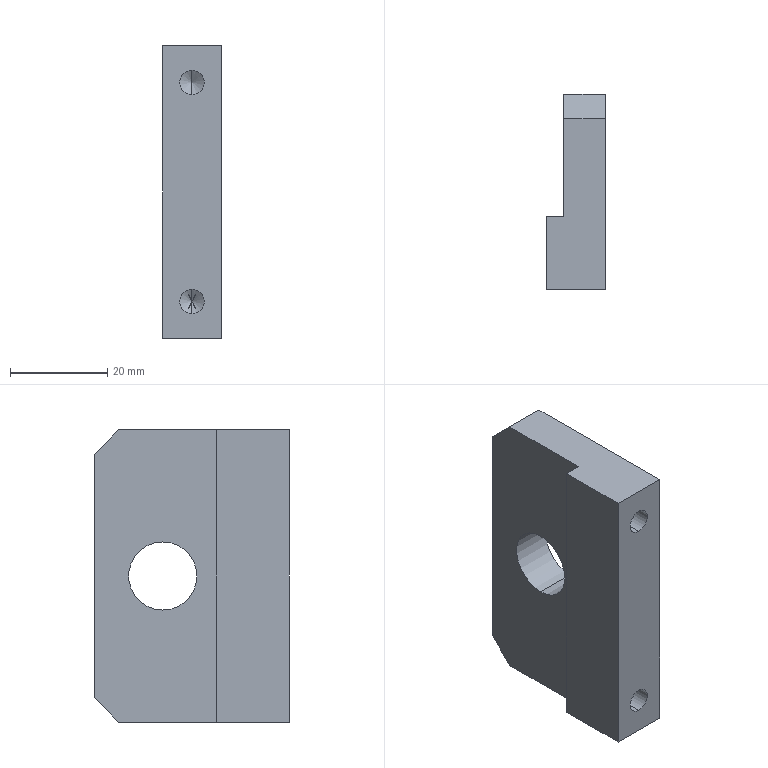Component | SolidWorks | OT-0100-009(TrunnionSeat)-1 | 1 solid | 20 faces | box 12 x 40 x 60 mm | volume 21499 mm3 | plane 10 | cylinder 6 | cone 4 | commonest cylinder face diameters 5 x4 14 x2 | material Plain Carbon Steel
build123d program:
from build123d import *

# Parameters (mm, degrees)
SKETCH1_W             = 60
SKETCH1_H             = 40
SKETCH1_R             = 7
BOSS_EXTRUDE1_DEPTH   = 6
M6_TAPPED_HOLE1_D     = 5
M6_TAPPED_HOLE1_DEPTH = 13
M6_TAPPED_HOLE1_TIP   = 1.502
SKETCH6_W             = 60
SKETCH6_H             = 25
CUT_EXTRUDE1_DEPTH    = 3.5
CHAMFER1_SIZE         = 5


with BuildPart() as part:
    # Sketch1 → Boss-Extrude1 (new, symmetric)
    with BuildSketch(Plane(origin=(0, 0, 0), x_dir=(0, 0, -1), z_dir=(1, 0, 0))):
        with Locations((0, 20)):
            Rectangle(SKETCH1_W, SKETCH1_H)
        with Locations((0, 26)):
            Circle(SKETCH1_R, mode=Mode.SUBTRACT)
    extrude(amount=BOSS_EXTRUDE1_DEPTH, both=True)

    # M6 Tapped Hole1
    with Locations(Plane(origin=(0, 0, 0), x_dir=(-1, 0, 0), z_dir=(0, -1, 0))):
        with Locations((0, -22.5), (0, 22.5)):
            Hole(M6_TAPPED_HOLE1_D / 2, depth=M6_TAPPED_HOLE1_DEPTH)
            with Locations((0, 0, -(M6_TAPPED_HOLE1_DEPTH + M6_TAPPED_HOLE1_TIP / 2))):  # 118° drill point
                Cone(0, M6_TAPPED_HOLE1_D / 2, M6_TAPPED_HOLE1_TIP, mode=Mode.SUBTRACT)

    # Sketch6 → Cut-Extrude1 (cut)
    with BuildSketch(Plane(origin=(-6, 0, 0), x_dir=(0, 0, -1), z_dir=(1, 0, 0))):
        with Locations((0, 27.5)):
            Rectangle(SKETCH6_W, SKETCH6_H)
    extrude(amount=CUT_EXTRUDE1_DEPTH, mode=Mode.SUBTRACT)

    # Chamfer1
    chamfer1_edges = [part.edges().sort_by_distance(p)[0] for p in [
        (1.75, 40, 30),
        (1.75, 40, -30),
    ]]
    chamfer(chamfer1_edges, length=CHAMFER1_SIZE)


solid = part.part

# Placed as in the assembly
solid = solid.moved(Location((170, 80, 100.5), (0, 0, 0)))
STEP:
#1=COLOUR_RGB('',0.7922,0.8196,0.9333);
#2=FILL_AREA_STYLE_COLOUR('',#1);
#3=FILL_AREA_STYLE('',(#2));
#4=SURFACE_STYLE_FILL_AREA(#3);
#5=SURFACE_SIDE_STYLE('',(#4));
#6=SURFACE_STYLE_USAGE(.BOTH.,#5);
#7=PRESENTATION_STYLE_ASSIGNMENT((#6));
#8=CARTESIAN_POINT('',(6.693,3.661,4.941));
#9=VERTEX_POINT('',#8);
#10=CARTESIAN_POINT('',(6.693,3.661,4.744));
#11=VERTEX_POINT('',#10);
#12=CARTESIAN_POINT('',(6.693,3.661,4.843));
#13=DIRECTION('',(0.,-1.,0.));
#14=DIRECTION('',(0.,0.,-1.));
#15=AXIS2_PLACEMENT_3D('',#12,#13,#14);
#16=CIRCLE('',#15,0.09843);
#17=EDGE_CURVE('',#9,#11,#16,.T.);
#18=ORIENTED_EDGE('',*,*,#17,.F.);
#19=CARTESIAN_POINT('',(6.693,3.15,4.941));
#20=VERTEX_POINT('',#19);
#21=CARTESIAN_POINT('',(6.693,3.15,4.941));
#22=DIRECTION('',(0.,-1.,0.));
#23=VECTOR('',#22,39.37);
#24=LINE('',#21,#23);
#25=EDGE_CURVE('',#9,#20,#24,.T.);
#26=ORIENTED_EDGE('',*,*,#25,.T.);
#27=CARTESIAN_POINT('',(6.693,3.15,4.744));
#28=VERTEX_POINT('',#27);
#29=CARTESIAN_POINT('',(6.693,3.15,4.843));
#30=DIRECTION('',(0.,-1.,0.));
#31=DIRECTION('',(0.,0.,-1.));
#32=AXIS2_PLACEMENT_3D('',#29,#30,#31);
#33=CIRCLE('',#32,0.09843);
#34=EDGE_CURVE('',#20,#28,#33,.T.);
#35=ORIENTED_EDGE('',*,*,#34,.T.);
#36=CARTESIAN_POINT('',(6.693,3.15,4.744));
#37=DIRECTION('',(0.,-1.,0.));
#38=VECTOR('',#37,39.37);
#39=LINE('',#36,#38);
#40=EDGE_CURVE('',#11,#28,#39,.T.);
#41=ORIENTED_EDGE('',*,*,#40,.F.);
#42=EDGE_LOOP('',(#18,#26,#35,#41));
#43=FACE_OUTER_BOUND('',#42,.T.);
#44=CARTESIAN_POINT('',(6.693,3.15,4.843));
#45=DIRECTION('',(0.,-1.,0.));
#46=DIRECTION('',(0.,0.,-1.));
#47=AXIS2_PLACEMENT_3D('',#44,#45,#46);
#48=CYLINDRICAL_SURFACE('',#47,0.09843);
#49=ADVANCED_FACE('',(#43),#48,.F.);
#50=CARTESIAN_POINT('',(6.693,3.721,4.843));
#51=VERTEX_POINT('',#50);
#52=CARTESIAN_POINT('',(6.693,3.661,4.744));
#53=DIRECTION('',(0.,-0.515,-0.8572));
#54=VECTOR('',#53,39.37);
#55=LINE('',#52,#54);
#56=EDGE_CURVE('',#51,#11,#55,.T.);
#57=ORIENTED_EDGE('',*,*,#56,.F.);
#58=CARTESIAN_POINT('',(6.693,3.661,4.941));
#59=DIRECTION('',(0.,-0.515,0.8572));
#60=VECTOR('',#59,39.37);
#61=LINE('',#58,#60);
#62=EDGE_CURVE('',#51,#9,#61,.T.);
#63=ORIENTED_EDGE('',*,*,#62,.T.);
#64=ORIENTED_EDGE('',*,*,#17,.T.);
#65=EDGE_LOOP('',(#57,#63,#64));
#66=FACE_OUTER_BOUND('',#65,.T.);
#67=CARTESIAN_POINT('',(6.693,3.661,4.843));
#68=DIRECTION('',(0.,-1.,0.));
#69=DIRECTION('',(0.,0.,-1.));
#70=AXIS2_PLACEMENT_3D('',#67,#68,#69);
#71=CONICAL_SURFACE('',#70,0.09843,1.03);
#72=ADVANCED_FACE('',(#66),#71,.F.);
#73=CARTESIAN_POINT('',(6.693,3.661,3.169));
#74=VERTEX_POINT('',#73);
#75=CARTESIAN_POINT('',(6.693,3.661,2.972));
#76=VERTEX_POINT('',#75);
#77=CARTESIAN_POINT('',(6.693,3.661,3.071));
#78=DIRECTION('',(0.,-1.,0.));
#79=DIRECTION('',(0.,0.,-1.));
#80=AXIS2_PLACEMENT_3D('',#77,#78,#79);
#81=CIRCLE('',#80,0.09843);
#82=EDGE_CURVE('',#74,#76,#81,.T.);
#83=ORIENTED_EDGE('',*,*,#82,.F.);
#84=CARTESIAN_POINT('',(6.693,3.15,3.169));
#85=VERTEX_POINT('',#84);
#86=CARTESIAN_POINT('',(6.693,3.15,3.169));
#87=DIRECTION('',(0.,-1.,0.));
#88=VECTOR('',#87,39.37);
#89=LINE('',#86,#88);
#90=EDGE_CURVE('',#74,#85,#89,.T.);
#91=ORIENTED_EDGE('',*,*,#90,.T.);
#92=CARTESIAN_POINT('',(6.693,3.15,2.972));
#93=VERTEX_POINT('',#92);
#94=CARTESIAN_POINT('',(6.693,3.15,3.071));
#95=DIRECTION('',(0.,-1.,0.));
#96=DIRECTION('',(0.,0.,-1.));
#97=AXIS2_PLACEMENT_3D('',#94,#95,#96);
#98=CIRCLE('',#97,0.09843);
#99=EDGE_CURVE('',#85,#93,#98,.T.);
#100=ORIENTED_EDGE('',*,*,#99,.T.);
#101=CARTESIAN_POINT('',(6.693,3.15,2.972));
#102=DIRECTION('',(0.,-1.,0.));
#103=VECTOR('',#102,39.37);
#104=LINE('',#101,#103);
#105=EDGE_CURVE('',#76,#93,#104,.T.);
#106=ORIENTED_EDGE('',*,*,#105,.F.);
#107=EDGE_LOOP('',(#83,#91,#100,#106));
#108=FACE_OUTER_BOUND('',#107,.T.);
#109=CARTESIAN_POINT('',(6.693,3.15,3.071));
#110=DIRECTION('',(0.,-1.,0.));
#111=DIRECTION('',(0.,0.,-1.));
#112=AXIS2_PLACEMENT_3D('',#109,#110,#111);
#113=CYLINDRICAL_SURFACE('',#112,0.09843);
#114=ADVANCED_FACE('',(#108),#113,.F.);
#115=CARTESIAN_POINT('',(6.693,3.721,3.071));
#116=VERTEX_POINT('',#115);
#117=CARTESIAN_POINT('',(6.693,3.661,2.972));
#118=DIRECTION('',(0.,-0.515,-0.8572));
#119=VECTOR('',#118,39.37);
#120=LINE('',#117,#119);
#121=EDGE_CURVE('',#116,#76,#120,.T.);
#122=ORIENTED_EDGE('',*,*,#121,.F.);
#123=CARTESIAN_POINT('',(6.693,3.661,3.169));
#124=DIRECTION('',(0.,-0.515,0.8572));
#125=VECTOR('',#124,39.37);
#126=LINE('',#123,#125);
#127=EDGE_CURVE('',#116,#74,#126,.T.);
#128=ORIENTED_EDGE('',*,*,#127,.T.);
#129=ORIENTED_EDGE('',*,*,#82,.T.);
#130=EDGE_LOOP('',(#122,#128,#129));
#131=FACE_OUTER_BOUND('',#130,.T.);
#132=CARTESIAN_POINT('',(6.693,3.661,3.071));
#133=DIRECTION('',(0.,-1.,0.));
#134=DIRECTION('',(0.,0.,-1.));
#135=AXIS2_PLACEMENT_3D('',#132,#133,#134);
#136=CONICAL_SURFACE('',#135,0.09843,1.03);
#137=ADVANCED_FACE('',(#131),#136,.F.);
#138=CARTESIAN_POINT('',(6.929,4.173,4.232));
#139=VERTEX_POINT('',#138);
#140=CARTESIAN_POINT('',(6.929,4.173,3.681));
#141=VERTEX_POINT('',#140);
#142=CARTESIAN_POINT('',(6.929,4.173,3.957));
#143=DIRECTION('',(1.,0.,0.));
#144=DIRECTION('',(0.,0.,-1.));
#145=AXIS2_PLACEMENT_3D('',#142,#143,#144);
#146=CIRCLE('',#145,0.2756);
#147=EDGE_CURVE('',#139,#141,#146,.T.);
#148=ORIENTED_EDGE('',*,*,#147,.T.);
#149=CARTESIAN_POINT('',(6.594,4.173,3.681));
#150=VERTEX_POINT('',#149);
#151=CARTESIAN_POINT('',(6.929,4.173,3.681));
#152=DIRECTION('',(-1.,0.,0.));
#153=VECTOR('',#152,39.37);
#154=LINE('',#151,#153);
#155=EDGE_CURVE('',#141,#150,#154,.T.);
#156=ORIENTED_EDGE('',*,*,#155,.T.);
#157=CARTESIAN_POINT('',(6.594,4.173,4.232));
#158=VERTEX_POINT('',#157);
#159=CARTESIAN_POINT('',(6.594,4.173,3.957));
#160=DIRECTION('',(1.,0.,0.));
#161=DIRECTION('',(0.,0.,-1.));
#162=AXIS2_PLACEMENT_3D('',#159,#160,#161);
#163=CIRCLE('',#162,0.2756);
#164=EDGE_CURVE('',#158,#150,#163,.T.);
#165=ORIENTED_EDGE('',*,*,#164,.F.);
#166=CARTESIAN_POINT('',(6.929,4.173,4.232));
#167=DIRECTION('',(-1.,0.,0.));
#168=VECTOR('',#167,39.37);
#169=LINE('',#166,#168);
#170=EDGE_CURVE('',#139,#158,#169,.T.);
#171=ORIENTED_EDGE('',*,*,#170,.F.);
#172=EDGE_LOOP('',(#148,#156,#165,#171));
#173=FACE_OUTER_BOUND('',#172,.T.);
#174=CARTESIAN_POINT('',(6.929,4.173,3.957));
#175=DIRECTION('',(-1.,0.,0.));
#176=DIRECTION('',(0.,0.,1.));
#177=AXIS2_PLACEMENT_3D('',#174,#175,#176);
#178=CYLINDRICAL_SURFACE('',#177,0.2756);
#179=ADVANCED_FACE('',(#173),#178,.F.);
#180=CARTESIAN_POINT('',(6.457,3.74,5.138));
#181=VERTEX_POINT('',#180);
#182=CARTESIAN_POINT('',(6.457,3.15,5.138));
#183=VERTEX_POINT('',#182);
#184=CARTESIAN_POINT('',(6.457,3.15,5.138));
#185=DIRECTION('',(0.,-1.,0.));
#186=VECTOR('',#185,39.37);
#187=LINE('',#184,#186);
#188=EDGE_CURVE('',#181,#183,#187,.T.);
#189=ORIENTED_EDGE('',*,*,#188,.F.);
#190=CARTESIAN_POINT('',(6.457,3.74,2.776));
#191=VERTEX_POINT('',#190);
#192=CARTESIAN_POINT('',(6.457,3.74,5.138));
#193=DIRECTION('',(0.,0.,-1.));
#194=VECTOR('',#193,39.37);
#195=LINE('',#192,#194);
#196=EDGE_CURVE('',#181,#191,#195,.T.);
#197=ORIENTED_EDGE('',*,*,#196,.T.);
#198=CARTESIAN_POINT('',(6.457,3.15,2.776));
#199=VERTEX_POINT('',#198);
#200=CARTESIAN_POINT('',(6.457,3.15,2.776));
#201=DIRECTION('',(0.,1.,0.));
#202=VECTOR('',#201,39.37);
#203=LINE('',#200,#202);
#204=EDGE_CURVE('',#199,#191,#203,.T.);
#205=ORIENTED_EDGE('',*,*,#204,.F.);
#206=CARTESIAN_POINT('',(6.457,3.15,5.138));
#207=DIRECTION('',(0.,0.,-1.));
#208=VECTOR('',#207,39.37);
#209=LINE('',#206,#208);
#210=EDGE_CURVE('',#183,#199,#209,.T.);
#211=ORIENTED_EDGE('',*,*,#210,.F.);
#212=EDGE_LOOP('',(#189,#197,#205,#211));
#213=FACE_OUTER_BOUND('',#212,.T.);
#214=CARTESIAN_POINT('',(6.457,3.15,3.957));
#215=DIRECTION('',(-1.,0.,0.));
#216=DIRECTION('',(0.,0.,1.));
#217=AXIS2_PLACEMENT_3D('',#214,#215,#216);
#218=PLANE('',#217);
#219=ADVANCED_FACE('',(#213),#218,.T.);
#220=CARTESIAN_POINT('',(6.929,4.528,5.138));
#221=VERTEX_POINT('',#220);
#222=CARTESIAN_POINT('',(6.929,3.15,5.138));
#223=VERTEX_POINT('',#222);
#224=CARTESIAN_POINT('',(6.929,3.15,5.138));
#225=DIRECTION('',(0.,-1.,0.));
#226=VECTOR('',#225,39.37);
#227=LINE('',#224,#226);
#228=EDGE_CURVE('',#221,#223,#227,.T.);
#229=ORIENTED_EDGE('',*,*,#228,.F.);
#230=CARTESIAN_POINT('',(6.594,4.528,5.138));
#231=VERTEX_POINT('',#230);
#232=CARTESIAN_POINT('',(6.929,4.528,5.138));
#233=DIRECTION('',(-1.,0.,0.));
#234=VECTOR('',#233,39.37);
#235=LINE('',#232,#234);
#236=EDGE_CURVE('',#221,#231,#235,.T.);
#237=ORIENTED_EDGE('',*,*,#236,.T.);
#238=CARTESIAN_POINT('',(6.594,3.74,5.138));
#239=VERTEX_POINT('',#238);
#240=CARTESIAN_POINT('',(6.594,4.724,5.138));
#241=DIRECTION('',(0.,-1.,-0.));
#242=VECTOR('',#241,39.37);
#243=LINE('',#240,#242);
#244=EDGE_CURVE('',#231,#239,#243,.T.);
#245=ORIENTED_EDGE('',*,*,#244,.T.);
#246=CARTESIAN_POINT('',(6.594,3.74,5.138));
#247=DIRECTION('',(-1.,0.,0.));
#248=VECTOR('',#247,39.37);
#249=LINE('',#246,#248);
#250=EDGE_CURVE('',#239,#181,#249,.T.);
#251=ORIENTED_EDGE('',*,*,#250,.T.);
#252=ORIENTED_EDGE('',*,*,#188,.T.);
#253=CARTESIAN_POINT('',(6.929,3.15,5.138));
#254=DIRECTION('',(-1.,0.,0.));
#255=VECTOR('',#254,39.37);
#256=LINE('',#253,#255);
#257=EDGE_CURVE('',#223,#183,#256,.T.);
#258=ORIENTED_EDGE('',*,*,#257,.F.);
#259=EDGE_LOOP('',(#229,#237,#245,#251,#252,#258));
#260=FACE_OUTER_BOUND('',#259,.T.);
#261=CARTESIAN_POINT('',(6.929,3.15,5.138));
#262=DIRECTION('',(0.,0.,-1.));
#263=DIRECTION('',(-1.,0.,0.));
#264=AXIS2_PLACEMENT_3D('',#261,#262,#263);
#265=PLANE('',#264);
#266=ADVANCED_FACE('',(#260),#265,.F.);
#267=CARTESIAN_POINT('',(6.594,3.74,2.776));
#268=VERTEX_POINT('',#267);
#269=CARTESIAN_POINT('',(6.594,4.528,2.776));
#270=VERTEX_POINT('',#269);
#271=CARTESIAN_POINT('',(6.594,4.724,2.776));
#272=DIRECTION('',(0.,1.,0.));
#273=VECTOR('',#272,39.37);
#274=LINE('',#271,#273);
#275=EDGE_CURVE('',#268,#270,#274,.T.);
#276=ORIENTED_EDGE('',*,*,#275,.T.);
#277=CARTESIAN_POINT('',(6.929,4.528,2.776));
#278=VERTEX_POINT('',#277);
#279=CARTESIAN_POINT('',(6.929,4.528,2.776));
#280=DIRECTION('',(1.,0.,0.));
#281=VECTOR('',#280,39.37);
#282=LINE('',#279,#281);
#283=EDGE_CURVE('',#270,#278,#282,.T.);
#284=ORIENTED_EDGE('',*,*,#283,.T.);
#285=CARTESIAN_POINT('',(6.929,3.15,2.776));
#286=VERTEX_POINT('',#285);
#287=CARTESIAN_POINT('',(6.929,3.15,2.776));
#288=DIRECTION('',(0.,1.,0.));
#289=VECTOR('',#288,39.37);
#290=LINE('',#287,#289);
#291=EDGE_CURVE('',#286,#278,#290,.T.);
#292=ORIENTED_EDGE('',*,*,#291,.F.);
#293=CARTESIAN_POINT('',(6.929,3.15,2.776));
#294=DIRECTION('',(-1.,0.,0.));
#295=VECTOR('',#294,39.37);
#296=LINE('',#293,#295);
#297=EDGE_CURVE('',#286,#199,#296,.T.);
#298=ORIENTED_EDGE('',*,*,#297,.T.);
#299=ORIENTED_EDGE('',*,*,#204,.T.);
#300=CARTESIAN_POINT('',(6.594,3.74,2.776));
#301=DIRECTION('',(-1.,0.,0.));
#302=VECTOR('',#301,39.37);
#303=LINE('',#300,#302);
#304=EDGE_CURVE('',#268,#191,#303,.T.);
#305=ORIENTED_EDGE('',*,*,#304,.F.);
#306=EDGE_LOOP('',(#276,#284,#292,#298,#299,#305));
#307=FACE_OUTER_BOUND('',#306,.T.);
#308=CARTESIAN_POINT('',(6.929,3.15,2.776));
#309=DIRECTION('',(0.,0.,1.));
#310=DIRECTION('',(1.,0.,0.));
#311=AXIS2_PLACEMENT_3D('',#308,#309,#310);
#312=PLANE('',#311);
#313=ADVANCED_FACE('',(#307),#312,.F.);
#314=CARTESIAN_POINT('',(6.929,4.724,2.972));
#315=VERTEX_POINT('',#314);
#316=CARTESIAN_POINT('',(6.929,4.724,4.941));
#317=VERTEX_POINT('',#316);
#318=CARTESIAN_POINT('',(6.929,4.724,5.138));
#319=DIRECTION('',(0.,0.,1.));
#320=VECTOR('',#319,39.37);
#321=LINE('',#318,#320);
#322=EDGE_CURVE('',#315,#317,#321,.T.);
#323=ORIENTED_EDGE('',*,*,#322,.T.);
#324=CARTESIAN_POINT('',(6.929,4.528,5.138));
#325=DIRECTION('',(0.,-0.7071,0.7071));
#326=VECTOR('',#325,39.37);
#327=LINE('',#324,#326);
#328=EDGE_CURVE('',#317,#221,#327,.T.);
#329=ORIENTED_EDGE('',*,*,#328,.T.);
#330=ORIENTED_EDGE('',*,*,#228,.T.);
#331=CARTESIAN_POINT('',(6.929,3.15,5.138));
#332=DIRECTION('',(0.,0.,-1.));
#333=VECTOR('',#332,39.37);
#334=LINE('',#331,#333);
#335=EDGE_CURVE('',#223,#286,#334,.T.);
#336=ORIENTED_EDGE('',*,*,#335,.T.);
#337=ORIENTED_EDGE('',*,*,#291,.T.);
#338=CARTESIAN_POINT('',(6.929,4.724,2.972));
#339=DIRECTION('',(0.,0.7071,0.7071));
#340=VECTOR('',#339,39.37);
#341=LINE('',#338,#340);
#342=EDGE_CURVE('',#278,#315,#341,.T.);
#343=ORIENTED_EDGE('',*,*,#342,.T.);
#344=EDGE_LOOP('',(#323,#329,#330,#336,#337,#343));
#345=FACE_OUTER_BOUND('',#344,.T.);
#346=ORIENTED_EDGE('',*,*,#147,.F.);
#347=CARTESIAN_POINT('',(6.929,4.173,3.957));
#348=DIRECTION('',(1.,0.,0.));
#349=DIRECTION('',(0.,0.,-1.));
#350=AXIS2_PLACEMENT_3D('',#347,#348,#349);
#351=CIRCLE('',#350,0.2756);
#352=EDGE_CURVE('',#141,#139,#351,.T.);
#353=ORIENTED_EDGE('',*,*,#352,.F.);
#354=EDGE_LOOP('',(#346,#353));
#355=FACE_BOUND('',#354,.T.);
#356=CARTESIAN_POINT('',(6.929,3.15,3.957));
#357=DIRECTION('',(-1.,0.,0.));
#358=DIRECTION('',(0.,0.,1.));
#359=AXIS2_PLACEMENT_3D('',#356,#357,#358);
#360=PLANE('',#359);
#361=ADVANCED_FACE('',(#345,#355),#360,.F.);
#362=CARTESIAN_POINT('',(6.693,3.15,4.843));
#363=DIRECTION('',(0.,-1.,0.));
#364=DIRECTION('',(0.,0.,-1.));
#365=AXIS2_PLACEMENT_3D('',#362,#363,#364);
#366=CIRCLE('',#365,0.09843);
#367=EDGE_CURVE('',#28,#20,#366,.T.);
#368=ORIENTED_EDGE('',*,*,#367,.F.);
#369=ORIENTED_EDGE('',*,*,#34,.F.);
#370=EDGE_LOOP('',(#368,#369));
#371=FACE_BOUND('',#370,.T.);
#372=CARTESIAN_POINT('',(6.693,3.15,3.071));
#373=DIRECTION('',(0.,-1.,0.));
#374=DIRECTION('',(0.,0.,-1.));
#375=AXIS2_PLACEMENT_3D('',#372,#373,#374);
#376=CIRCLE('',#375,0.09843);
#377=EDGE_CURVE('',#93,#85,#376,.T.);
#378=ORIENTED_EDGE('',*,*,#377,.F.);
#379=ORIENTED_EDGE('',*,*,#99,.F.);
#380=EDGE_LOOP('',(#378,#379));
#381=FACE_BOUND('',#380,.T.);
#382=ORIENTED_EDGE('',*,*,#210,.T.);
#383=ORIENTED_EDGE('',*,*,#297,.F.);
#384=ORIENTED_EDGE('',*,*,#335,.F.);
#385=ORIENTED_EDGE('',*,*,#257,.T.);
#386=EDGE_LOOP('',(#382,#383,#384,#385));
#387=FACE_OUTER_BOUND('',#386,.T.);
#388=CARTESIAN_POINT('',(6.929,3.15,5.138));
#389=DIRECTION('',(0.,1.,0.));
#390=DIRECTION('',(0.,0.,1.));
#391=AXIS2_PLACEMENT_3D('',#388,#389,#390);
#392=PLANE('',#391);
#393=ADVANCED_FACE('',(#371,#381,#387),#392,.F.);
#394=CARTESIAN_POINT('',(6.594,4.724,2.972));
#395=VERTEX_POINT('',#394);
#396=CARTESIAN_POINT('',(6.594,4.724,4.941));
#397=VERTEX_POINT('',#396);
#398=CARTESIAN_POINT('',(6.594,4.724,5.138));
#399=DIRECTION('',(0.,0.,1.));
#400=VECTOR('',#399,39.37);
#401=LINE('',#398,#400);
#402=EDGE_CURVE('',#395,#397,#401,.T.);
#403=ORIENTED_EDGE('',*,*,#402,.T.);
#404=CARTESIAN_POINT('',(6.929,4.724,4.941));
#405=DIRECTION('',(1.,0.,0.));
#406=VECTOR('',#405,39.37);
#407=LINE('',#404,#406);
#408=EDGE_CURVE('',#397,#317,#407,.T.);
#409=ORIENTED_EDGE('',*,*,#408,.T.);
#410=ORIENTED_EDGE('',*,*,#322,.F.);
#411=CARTESIAN_POINT('',(6.929,4.724,2.972));
#412=DIRECTION('',(-1.,0.,0.));
#413=VECTOR('',#412,39.37);
#414=LINE('',#411,#413);
#415=EDGE_CURVE('',#315,#395,#414,.T.);
#416=ORIENTED_EDGE('',*,*,#415,.T.);
#417=EDGE_LOOP('',(#403,#409,#410,#416));
#418=FACE_OUTER_BOUND('',#417,.T.);
#419=CARTESIAN_POINT('',(6.929,4.724,5.138));
#420=DIRECTION('',(0.,-1.,0.));
#421=DIRECTION('',(0.,0.,-1.));
#422=AXIS2_PLACEMENT_3D('',#419,#420,#421);
#423=PLANE('',#422);
#424=ADVANCED_FACE('',(#418),#423,.F.);
#425=ORIENTED_EDGE('',*,*,#155,.F.);
#426=ORIENTED_EDGE('',*,*,#352,.T.);
#427=ORIENTED_EDGE('',*,*,#170,.T.);
#428=CARTESIAN_POINT('',(6.594,4.173,3.957));
#429=DIRECTION('',(1.,0.,0.));
#430=DIRECTION('',(0.,0.,-1.));
#431=AXIS2_PLACEMENT_3D('',#428,#429,#430);
#432=CIRCLE('',#431,0.2756);
#433=EDGE_CURVE('',#150,#158,#432,.T.);
#434=ORIENTED_EDGE('',*,*,#433,.F.);
#435=EDGE_LOOP('',(#425,#426,#427,#434));
#436=FACE_OUTER_BOUND('',#435,.T.);
#437=CARTESIAN_POINT('',(6.929,4.173,3.957));
#438=DIRECTION('',(-1.,0.,0.));
#439=DIRECTION('',(0.,0.,1.));
#440=AXIS2_PLACEMENT_3D('',#437,#438,#439);
#441=CYLINDRICAL_SURFACE('',#440,0.2756);
#442=ADVANCED_FACE('',(#436),#441,.F.);
#443=ORIENTED_EDGE('',*,*,#127,.F.);
#444=ORIENTED_EDGE('',*,*,#121,.T.);
#445=CARTESIAN_POINT('',(6.693,3.661,3.071));
#446=DIRECTION('',(0.,-1.,0.));
#447=DIRECTION('',(0.,0.,-1.));
#448=AXIS2_PLACEMENT_3D('',#445,#446,#447);
#449=CIRCLE('',#448,0.09843);
#450=EDGE_CURVE('',#76,#74,#449,.T.);
#451=ORIENTED_EDGE('',*,*,#450,.T.);
#452=EDGE_LOOP('',(#443,#444,#451));
#453=FACE_OUTER_BOUND('',#452,.T.);
#454=CARTESIAN_POINT('',(6.693,3.661,3.071));
#455=DIRECTION('',(0.,-1.,0.));
#456=DIRECTION('',(0.,0.,-1.));
#457=AXIS2_PLACEMENT_3D('',#454,#455,#456);
#458=CONICAL_SURFACE('',#457,0.09843,1.03);
#459=ADVANCED_FACE('',(#453),#458,.F.);
#460=ORIENTED_EDGE('',*,*,#90,.F.);
#461=ORIENTED_EDGE('',*,*,#450,.F.);
#462=ORIENTED_EDGE('',*,*,#105,.T.);
#463=ORIENTED_EDGE('',*,*,#377,.T.);
#464=EDGE_LOOP('',(#460,#461,#462,#463));
#465=FACE_OUTER_BOUND('',#464,.T.);
#466=CARTESIAN_POINT('',(6.693,3.15,3.071));
#467=DIRECTION('',(0.,-1.,0.));
#468=DIRECTION('',(0.,0.,-1.));
#469=AXIS2_PLACEMENT_3D('',#466,#467,#468);
#470=CYLINDRICAL_SURFACE('',#469,0.09843);
#471=ADVANCED_FACE('',(#465),#470,.F.);
#472=ORIENTED_EDGE('',*,*,#62,.F.);
#473=ORIENTED_EDGE('',*,*,#56,.T.);
#474=CARTESIAN_POINT('',(6.693,3.661,4.843));
#475=DIRECTION('',(0.,-1.,0.));
#476=DIRECTION('',(0.,0.,-1.));
#477=AXIS2_PLACEMENT_3D('',#474,#475,#476);
#478=CIRCLE('',#477,0.09843);
#479=EDGE_CURVE('',#11,#9,#478,.T.);
#480=ORIENTED_EDGE('',*,*,#479,.T.);
#481=EDGE_LOOP('',(#472,#473,#480));
#482=FACE_OUTER_BOUND('',#481,.T.);
#483=CARTESIAN_POINT('',(6.693,3.661,4.843));
#484=DIRECTION('',(0.,-1.,0.));
#485=DIRECTION('',(0.,0.,-1.));
#486=AXIS2_PLACEMENT_3D('',#483,#484,#485);
#487=CONICAL_SURFACE('',#486,0.09843,1.03);
#488=ADVANCED_FACE('',(#482),#487,.F.);
#489=ORIENTED_EDGE('',*,*,#25,.F.);
#490=ORIENTED_EDGE('',*,*,#479,.F.);
#491=ORIENTED_EDGE('',*,*,#40,.T.);
#492=ORIENTED_EDGE('',*,*,#367,.T.);
#493=EDGE_LOOP('',(#489,#490,#491,#492));
#494=FACE_OUTER_BOUND('',#493,.T.);
#495=CARTESIAN_POINT('',(6.693,3.15,4.843));
#496=DIRECTION('',(0.,-1.,0.));
#497=DIRECTION('',(0.,0.,-1.));
#498=AXIS2_PLACEMENT_3D('',#495,#496,#497);
#499=CYLINDRICAL_SURFACE('',#498,0.09843);
#500=ADVANCED_FACE('',(#494),#499,.F.);
#501=ORIENTED_EDGE('',*,*,#196,.F.);
#502=ORIENTED_EDGE('',*,*,#250,.F.);
#503=CARTESIAN_POINT('',(6.594,3.74,5.138));
#504=DIRECTION('',(0.,0.,-1.));
#505=VECTOR('',#504,39.37);
#506=LINE('',#503,#505);
#507=EDGE_CURVE('',#239,#268,#506,.T.);
#508=ORIENTED_EDGE('',*,*,#507,.T.);
#509=ORIENTED_EDGE('',*,*,#304,.T.);
#510=EDGE_LOOP('',(#501,#502,#508,#509));
#511=FACE_OUTER_BOUND('',#510,.T.);
#512=CARTESIAN_POINT('',(6.594,3.74,5.138));
#513=DIRECTION('',(0.,1.,0.));
#514=DIRECTION('',(0.,0.,1.));
#515=AXIS2_PLACEMENT_3D('',#512,#513,#514);
#516=PLANE('',#515);
#517=ADVANCED_FACE('',(#511),#516,.T.);
#518=ORIENTED_EDGE('',*,*,#164,.T.);
#519=ORIENTED_EDGE('',*,*,#433,.T.);
#520=EDGE_LOOP('',(#518,#519));
#521=FACE_BOUND('',#520,.T.);
#522=ORIENTED_EDGE('',*,*,#244,.F.);
#523=CARTESIAN_POINT('',(6.594,4.528,5.138));
#524=DIRECTION('',(0.,0.7071,-0.7071));
#525=VECTOR('',#524,39.37);
#526=LINE('',#523,#525);
#527=EDGE_CURVE('',#231,#397,#526,.T.);
#528=ORIENTED_EDGE('',*,*,#527,.T.);
#529=ORIENTED_EDGE('',*,*,#402,.F.);
#530=CARTESIAN_POINT('',(6.594,4.724,2.972));
#531=DIRECTION('',(0.,-0.7071,-0.7071));
#532=VECTOR('',#531,39.37);
#533=LINE('',#530,#532);
#534=EDGE_CURVE('',#395,#270,#533,.T.);
#535=ORIENTED_EDGE('',*,*,#534,.T.);
#536=ORIENTED_EDGE('',*,*,#275,.F.);
#537=ORIENTED_EDGE('',*,*,#507,.F.);
#538=EDGE_LOOP('',(#522,#528,#529,#535,#536,#537));
#539=FACE_OUTER_BOUND('',#538,.T.);
#540=CARTESIAN_POINT('',(6.594,3.15,3.957));
#541=DIRECTION('',(1.,0.,0.));
#542=DIRECTION('',(0.,0.,-1.));
#543=AXIS2_PLACEMENT_3D('',#540,#541,#542);
#544=PLANE('',#543);
#545=ADVANCED_FACE('',(#521,#539),#544,.F.);
#546=ORIENTED_EDGE('',*,*,#328,.F.);
#547=ORIENTED_EDGE('',*,*,#408,.F.);
#548=ORIENTED_EDGE('',*,*,#527,.F.);
#549=ORIENTED_EDGE('',*,*,#236,.F.);
#550=EDGE_LOOP('',(#546,#547,#548,#549));
#551=FACE_OUTER_BOUND('',#550,.T.);
#552=CARTESIAN_POINT('',(6.929,4.528,5.138));
#553=DIRECTION('',(0.,-0.7071,-0.7071));
#554=DIRECTION('',(-1.,0.,0.));
#555=AXIS2_PLACEMENT_3D('',#552,#553,#554);
#556=PLANE('',#555);
#557=ADVANCED_FACE('',(#551),#556,.F.);
#558=ORIENTED_EDGE('',*,*,#342,.F.);
#559=ORIENTED_EDGE('',*,*,#283,.F.);
#560=ORIENTED_EDGE('',*,*,#534,.F.);
#561=ORIENTED_EDGE('',*,*,#415,.F.);
#562=EDGE_LOOP('',(#558,#559,#560,#561));
#563=FACE_OUTER_BOUND('',#562,.T.);
#564=CARTESIAN_POINT('',(6.929,4.724,2.972));
#565=DIRECTION('',(0.,-0.7071,0.7071));
#566=DIRECTION('',(-1.,0.,0.));
#567=AXIS2_PLACEMENT_3D('',#564,#565,#566);
#568=PLANE('',#567);
#569=ADVANCED_FACE('',(#563),#568,.F.);
#570=CLOSED_SHELL('',(#49,#72,#114,#137,#179,#219,#266,#313,#361,#393,#424,#442,#459,#471,#488,#500,#517,#545,#557,#569));
#571=MANIFOLD_SOLID_BREP('',#570);
#572=STYLED_ITEM('',(#7),#571);
#573=PRESENTATION_LAYER_ASSIGNMENT('','',(#572));
#574=CARTESIAN_POINT('',(0.,0.,0.));
#575=DIRECTION('',(0.,0.,1.));
#576=DIRECTION('',(1.,0.,0.));
#577=AXIS2_PLACEMENT_3D('',#574,#575,#576);
#578=(LENGTH_UNIT()NAMED_UNIT(*)SI_UNIT($,.METRE.));
#579=LENGTH_MEASURE_WITH_UNIT(LENGTH_MEASURE(0.0254),#578);
#580=DIMENSIONAL_EXPONENTS(1.,0.,0.,0.,0.,0.,0.);
#581=(CONVERSION_BASED_UNIT('',#579)LENGTH_UNIT()NAMED_UNIT(#580));
#582=UNCERTAINTY_MEASURE_WITH_UNIT(LENGTH_MEASURE(0.00001),#581,'','');
#583=(NAMED_UNIT(*)PLANE_ANGLE_UNIT()SI_UNIT($,.RADIAN.));
#584=(NAMED_UNIT(*)SI_UNIT($,.STERADIAN.)SOLID_ANGLE_UNIT());
#585=(GEOMETRIC_REPRESENTATION_CONTEXT(3)GLOBAL_UNCERTAINTY_ASSIGNED_CONTEXT((#582))GLOBAL_UNIT_ASSIGNED_CONTEXT((#581,#583,#584))REPRESENTATION_CONTEXT('',''));
#586=ADVANCED_BREP_SHAPE_REPRESENTATION('',(#571,#577),#585);
#587=(LENGTH_UNIT()NAMED_UNIT(*)SI_UNIT($,.METRE.));
#588=LENGTH_MEASURE_WITH_UNIT(LENGTH_MEASURE(0.0254),#587);
#589=DIMENSIONAL_EXPONENTS(1.,0.,0.,0.,0.,0.,0.);
#590=(CONVERSION_BASED_UNIT('',#588)LENGTH_UNIT()NAMED_UNIT(#589));
#591=UNCERTAINTY_MEASURE_WITH_UNIT(LENGTH_MEASURE(0.00001),#590,'','');
#592=(NAMED_UNIT(*)PLANE_ANGLE_UNIT()SI_UNIT($,.RADIAN.));
#593=(NAMED_UNIT(*)SI_UNIT($,.STERADIAN.)SOLID_ANGLE_UNIT());
#594=(GEOMETRIC_REPRESENTATION_CONTEXT(3)GLOBAL_UNCERTAINTY_ASSIGNED_CONTEXT((#591))GLOBAL_UNIT_ASSIGNED_CONTEXT((#590,#592,#593))REPRESENTATION_CONTEXT('',''));
#595=MECHANICAL_DESIGN_GEOMETRIC_PRESENTATION_REPRESENTATION('',(#572),#594);